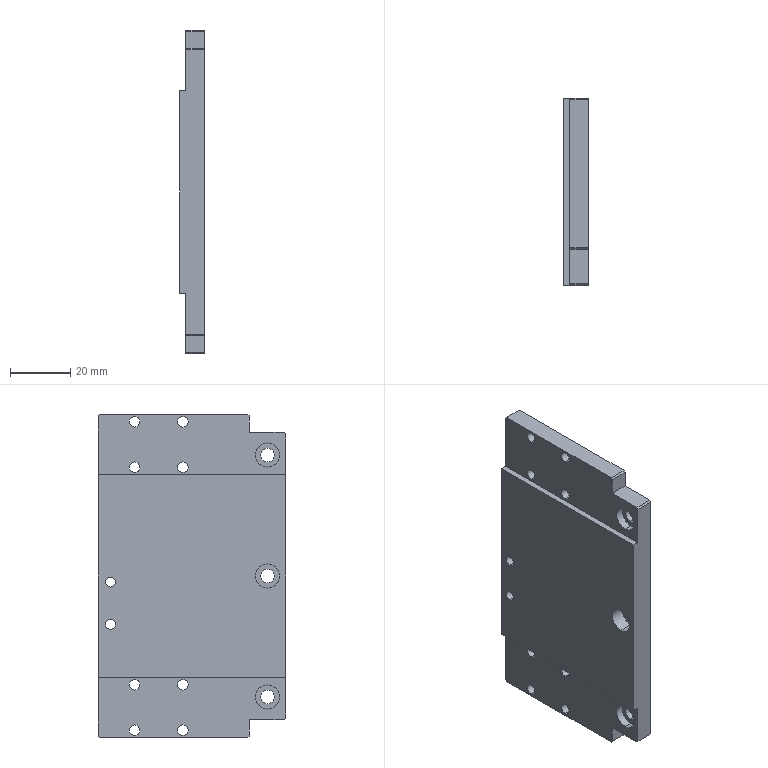Component | SolidWorks | F01AE00021-D54311-1 | 1 solid | 55 faces | volume 45990 mm3 | cylinder 32 | plane 23 | commonest cylinder face diameters 3.5 x16 8 x6 4.5 x6 3.3 x4